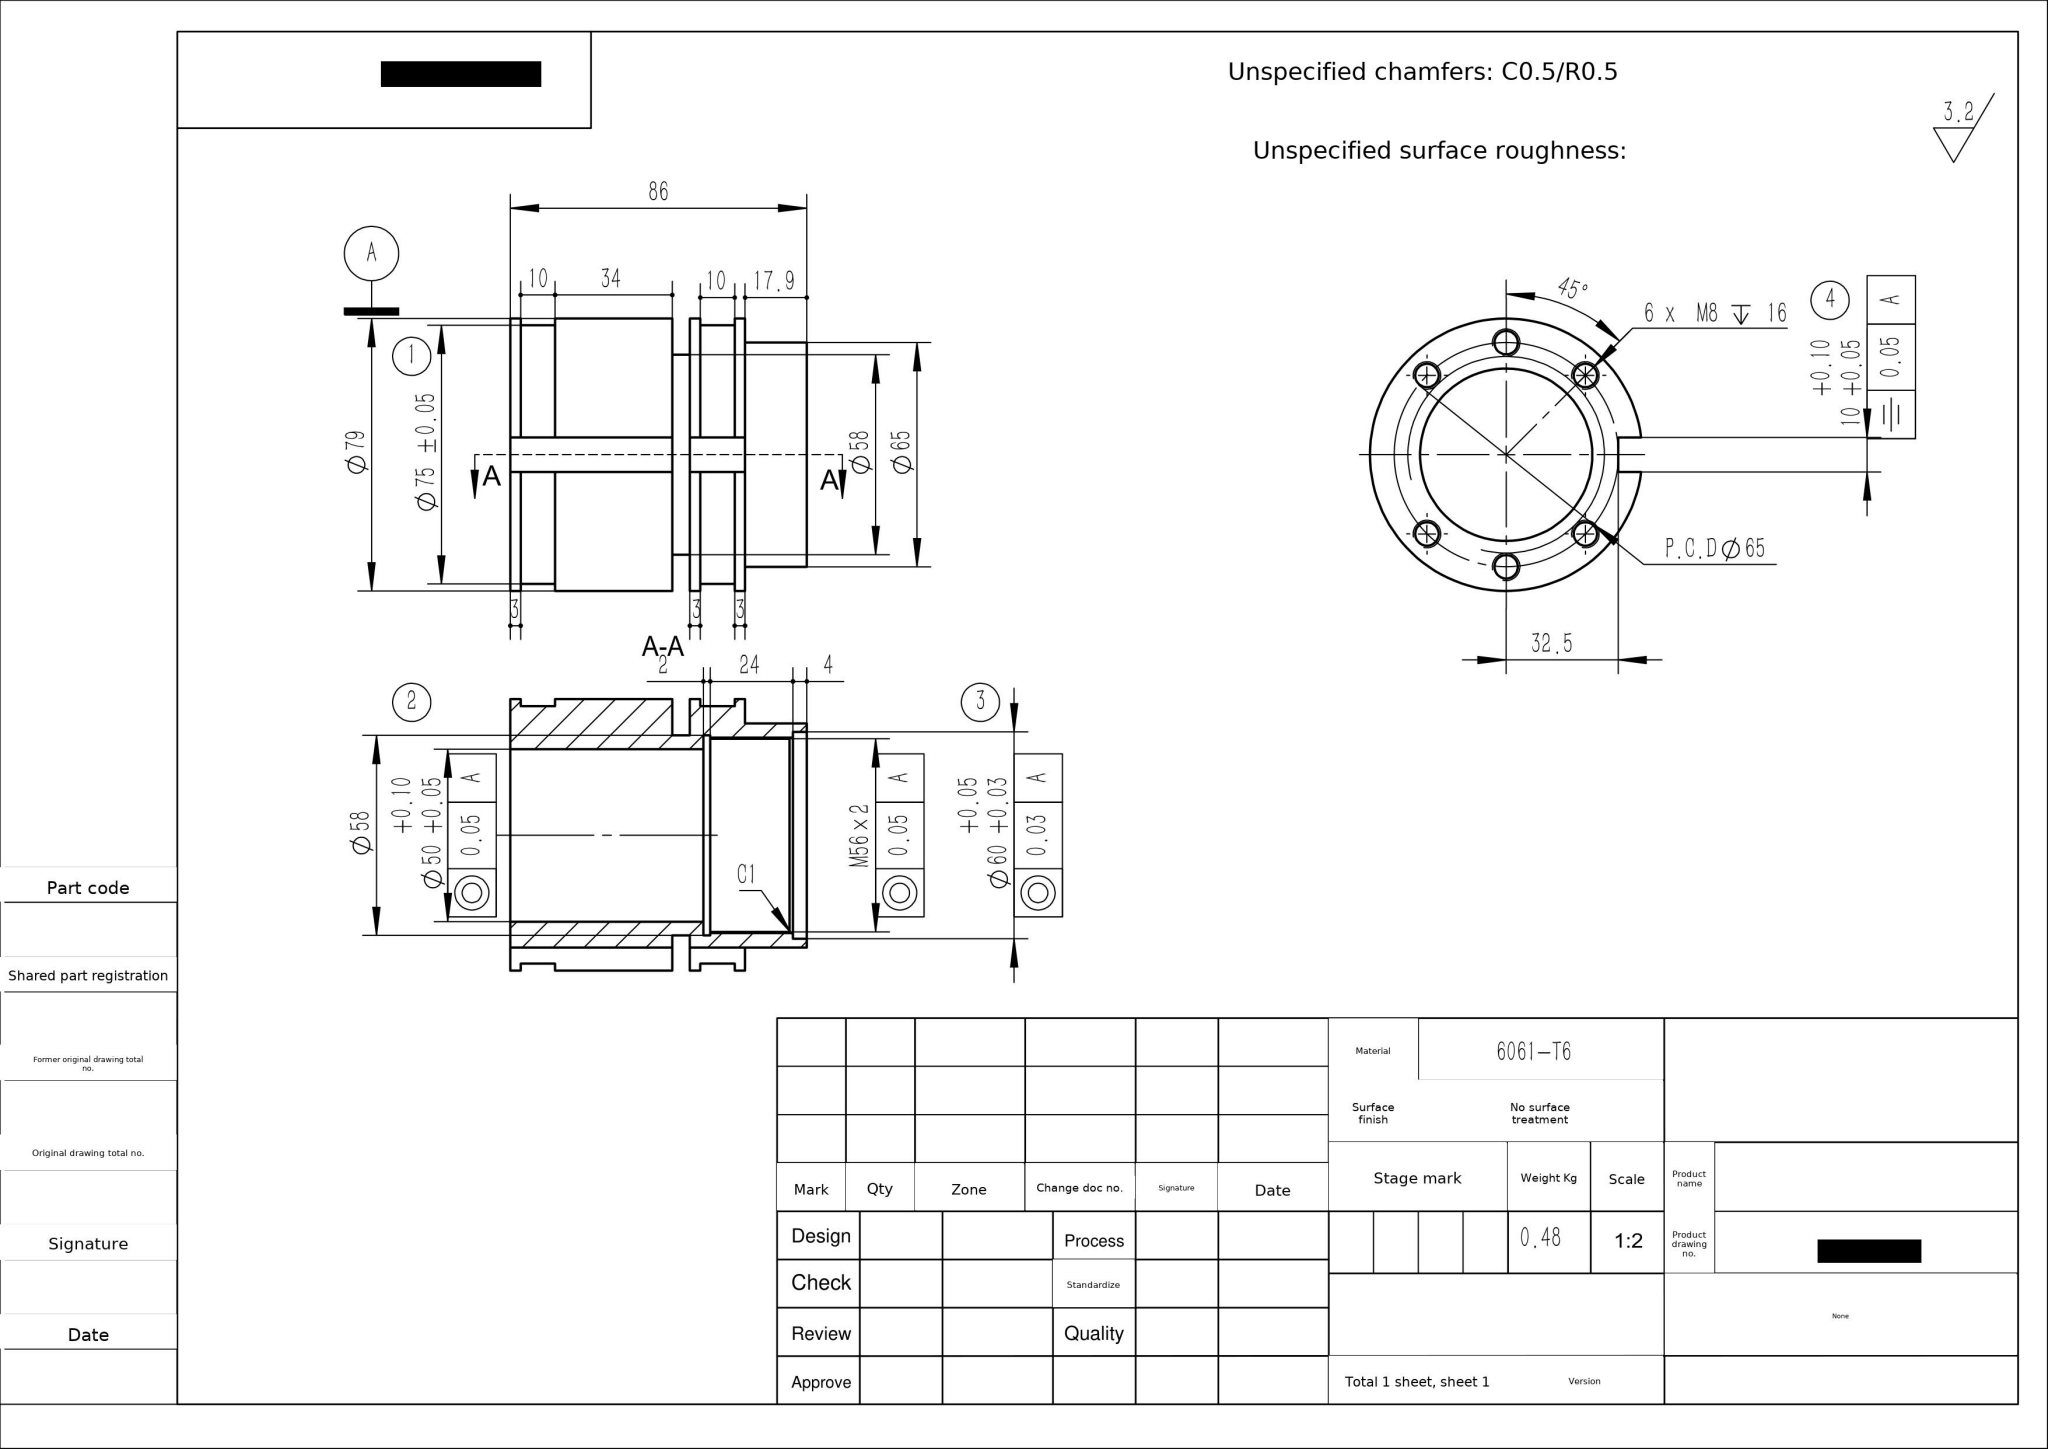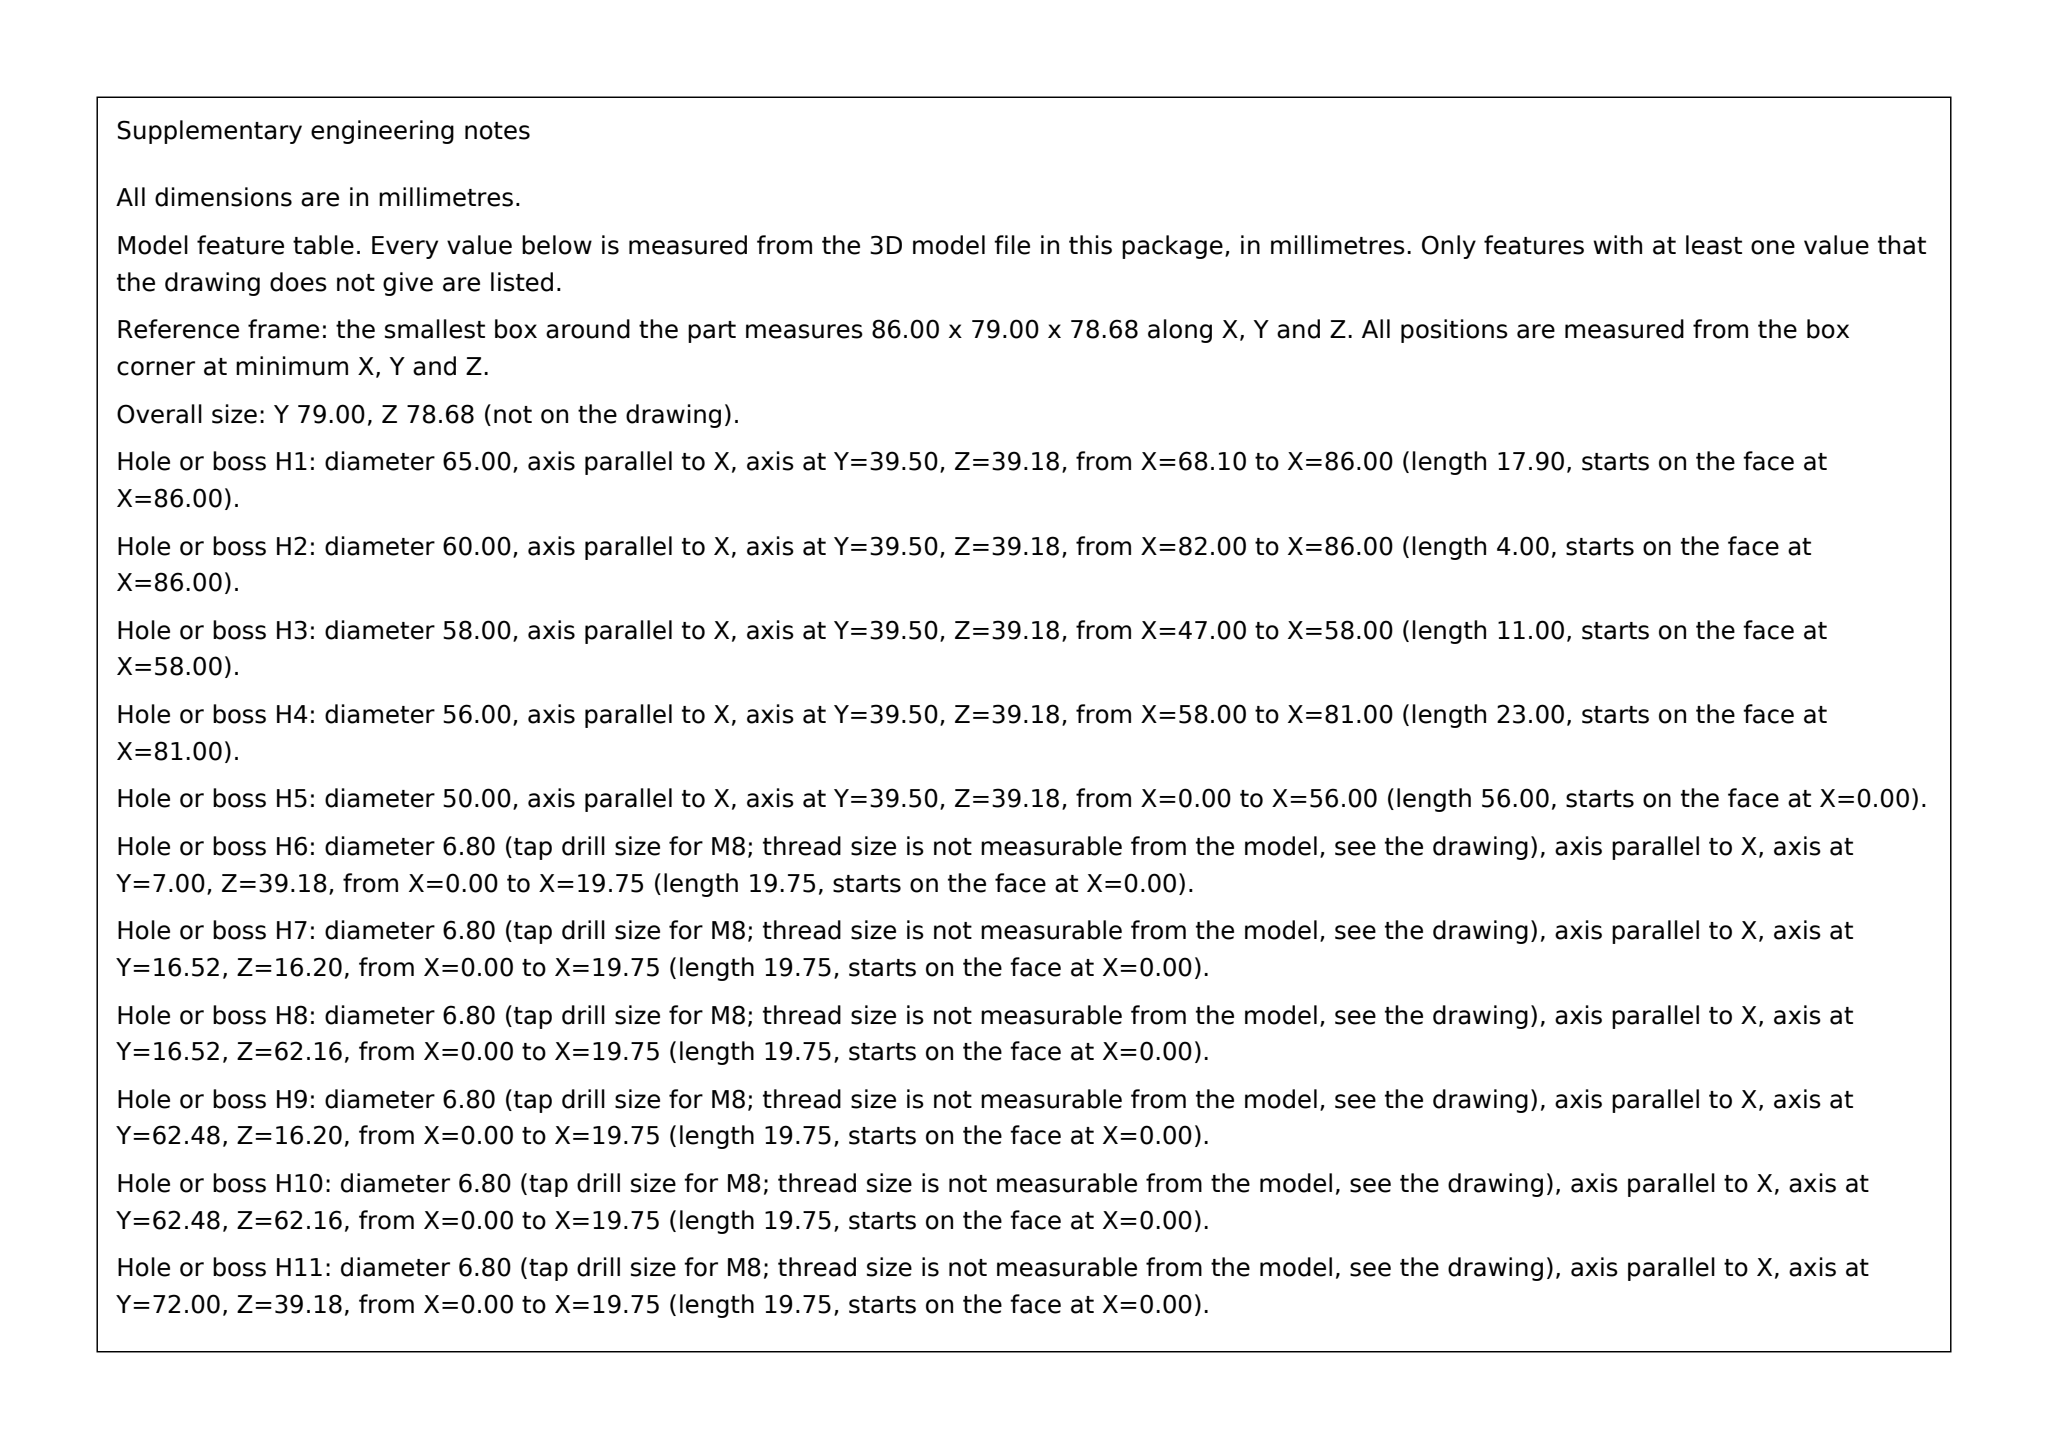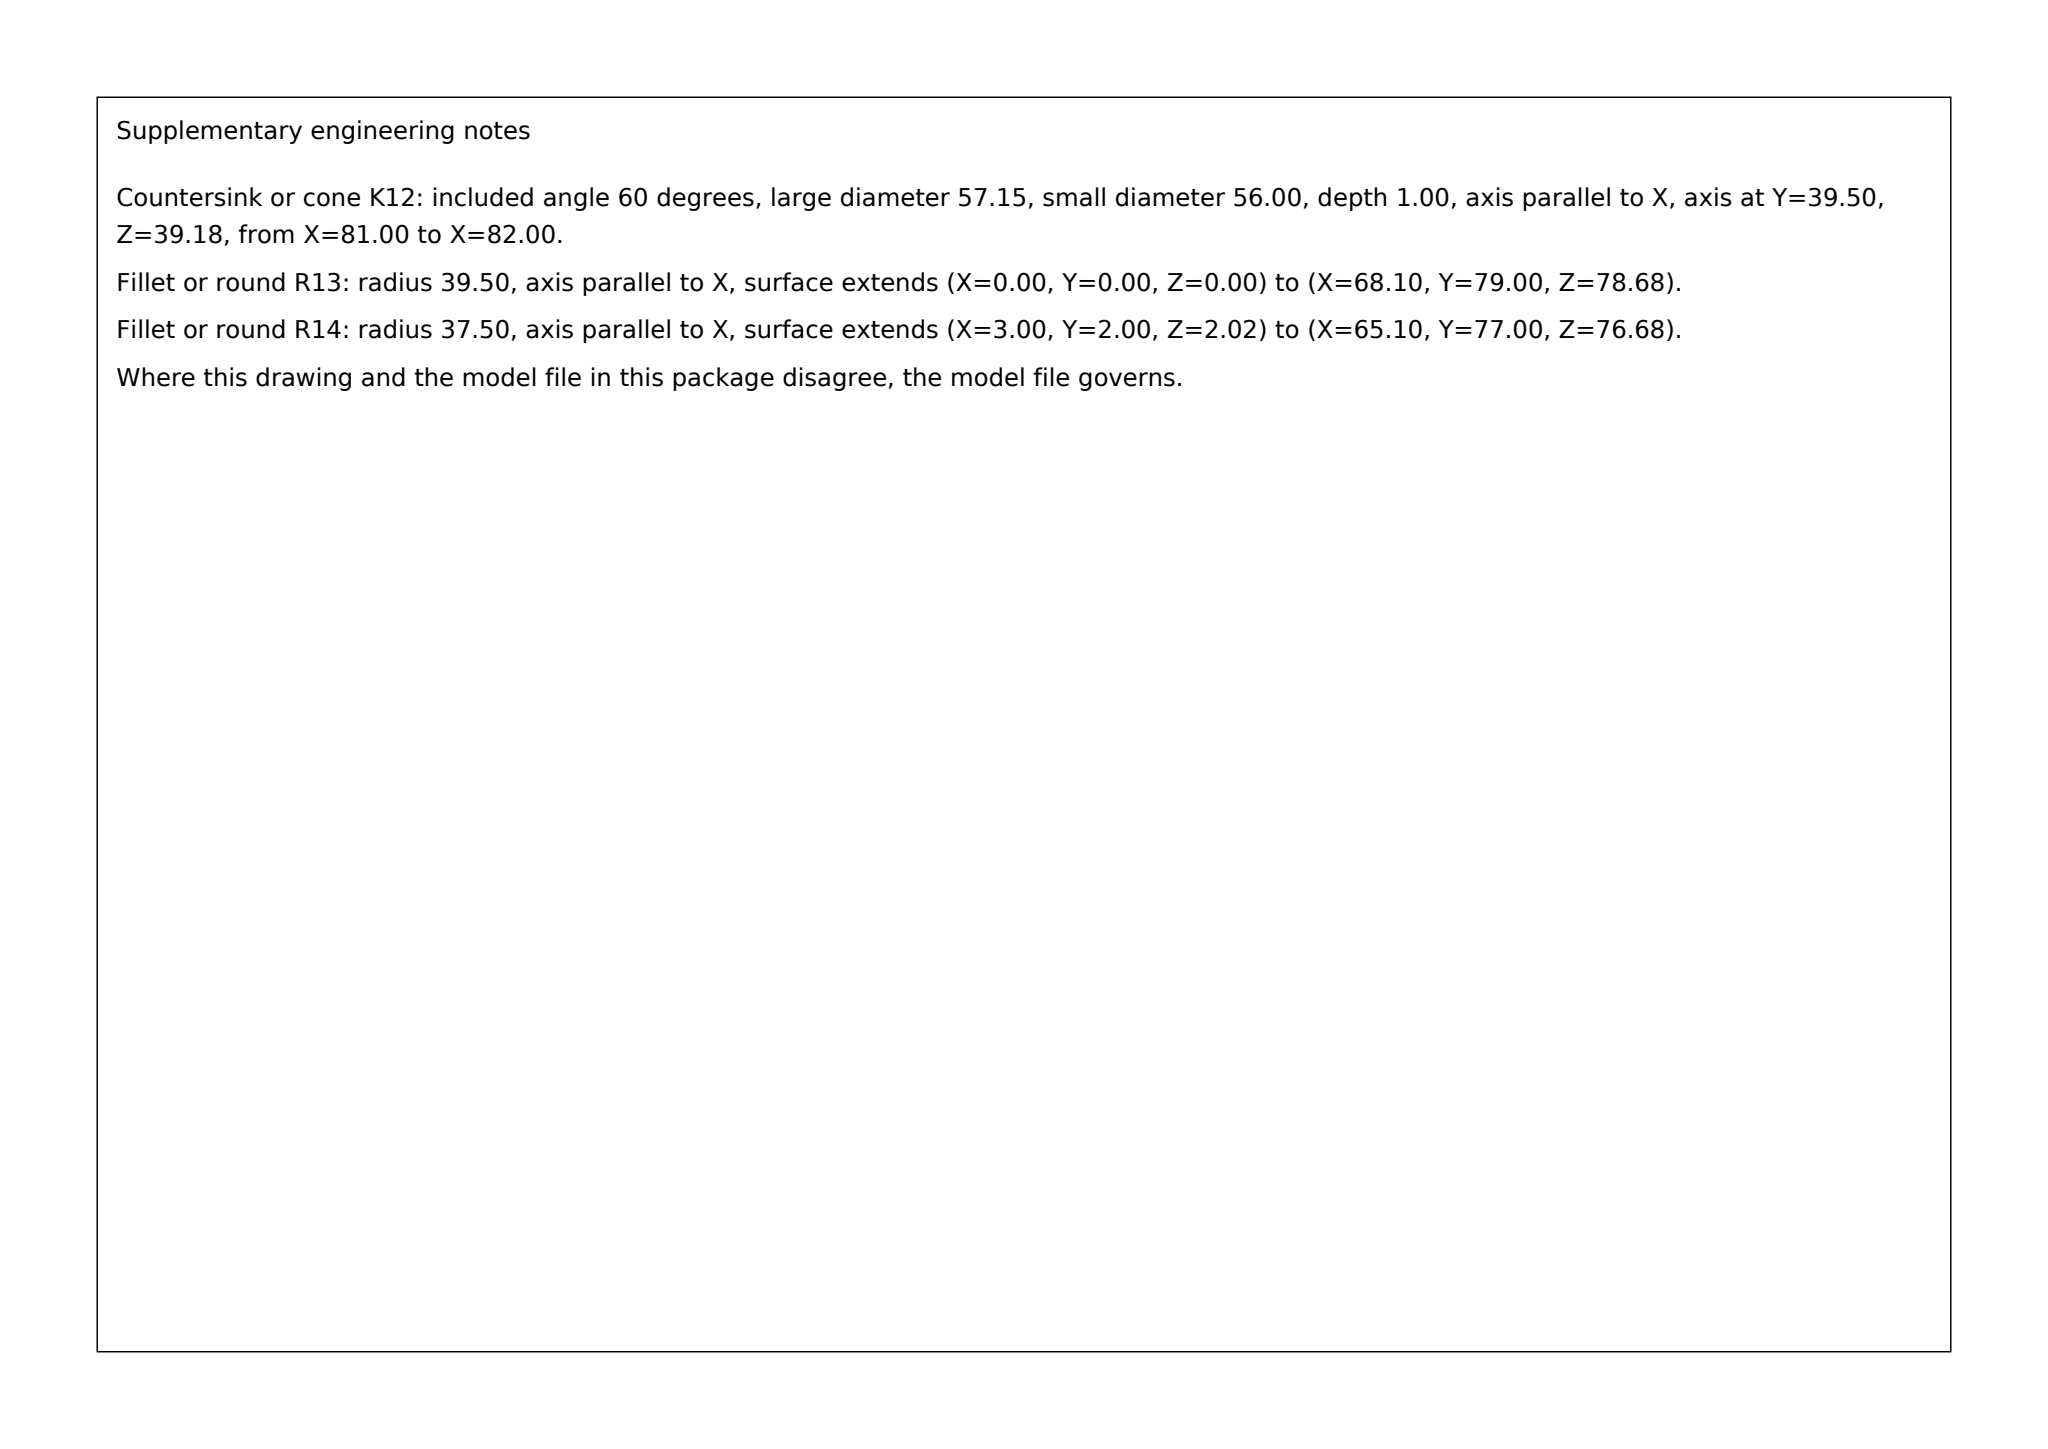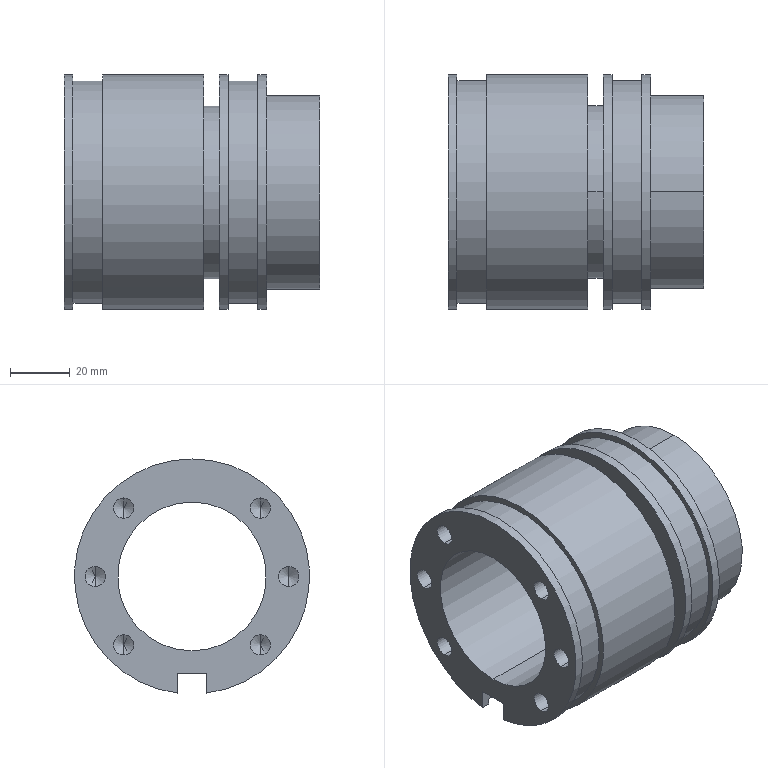Part | SolidWorks | mm | material 6061-T6 | 1 solid | 62 faces | box 86 x 79 x 78.68 mm | volume 177894 mm3 | cylinder 30 | plane 18 | cone 14 | commonest cylinder face diameters 6.8 x12 58 x4 79 x4 60 x2 56 x2 50 x2 65 x2 75 x2
build123d program:
from build123d import *

# Parameters (mm, degrees)
M8_TAPPED_HOLE1_D     = 6.8
M8_TAPPED_HOLE1_DEPTH = 19.75
M8_TAPPED_HOLE1_TIP   = 2.043
CUT_EXTRUDE2_START    = 2
SKETCH10_R            = 29
CUT_EXTRUDE2_DEPTH    = 2
SKETCH11_W            = 13.633
SKETCH11_H            = 10
CUT_EXTRUDE3_DEPTH    = 103.55


with BuildPart() as part:
    # Sketch2 → Revolve1 (revolve)
    with BuildSketch(Plane.XY, mode=Mode.PRIVATE) as revolve1_sk:
        Polygon((0, 0), (0, 39.5), (3, 39.5), (3, 37.5), (13, 37.5), (13, 39.5), (47, 39.5), (47, 29), (52.1, 29), (52.1, 39.5), (55.1, 39.5), (55.1, 37.5), (65.1, 37.5), (65.1, 39.5), (68.1, 39.5), (68.1, 32.5), (86, 32.5), (86, 0), align=None)
    revolve(revolve1_sk.sketch.rotate(Axis((86, 0, 0), (-1, 0, 0)), 90), axis=Axis((86, 0, 0), (-1, 0, 0)))

    # Sketch3 → Cut-Revolve1 (revolve, cut)
    with BuildSketch(Plane.XY, mode=Mode.PRIVATE) as cut_revolve1_sk:
        Polygon((0, 0), (0, 25), (56, 25), (56, 28), (81, 28), (82, 28.577), (82, 30), (86, 30), (86, 0), align=None)
    revolve(cut_revolve1_sk.sketch.rotate(Axis((86, 0, 0), (-1, 0, 0)), 90), axis=Axis((86, 0, 0), (-1, 0, 0)), mode=Mode.SUBTRACT)

    # M8 Tapped Hole1
    with Locations(Plane.ZY):
        with Locations((-22.981, 22.981), (22.981, -22.981), (22.981, 22.981), (-22.981, -22.981), (0, 32.5), (0, -32.5)):
            Hole(M8_TAPPED_HOLE1_D / 2, depth=M8_TAPPED_HOLE1_DEPTH)
            with Locations((0, 0, -(M8_TAPPED_HOLE1_DEPTH + M8_TAPPED_HOLE1_TIP / 2))):  # 118° drill point
                Cone(0, M8_TAPPED_HOLE1_D / 2, M8_TAPPED_HOLE1_TIP, mode=Mode.SUBTRACT)

    # Sketch10 → Cut-Extrude2 (cut)
    with BuildSketch(Plane(origin=(56, 0, 0), x_dir=(0, 0, -1), z_dir=(1, 0, 0)).offset(CUT_EXTRUDE2_START)):
        Circle(SKETCH10_R)
    extrude(amount=-CUT_EXTRUDE2_DEPTH, mode=Mode.SUBTRACT)

    # Sketch11 → Cut-Extrude3 (cut, through all)
    with BuildSketch(Plane.ZY):
        with Locations((-39.316, 0)):
            Rectangle(SKETCH11_W, SKETCH11_H)
    extrude(amount=-CUT_EXTRUDE3_DEPTH, mode=Mode.SUBTRACT)


solid = part.part